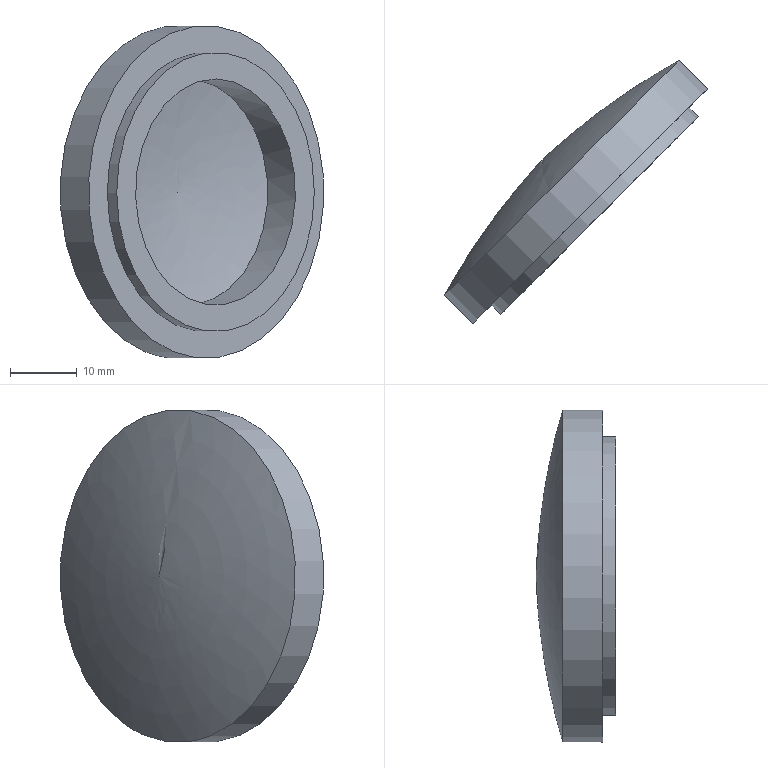Component | NX | END_CAP | 1 solid | 7 faces | box 39.6 x 39.6 x 50 mm | volume 12004 mm3 | cylinder 3 | plane 2 | spline 2 | commonest cylinder face diameters 42 x1 50 x1 34 x1
STEP:
#1=CARTESIAN_POINT('',(0.,0.,0.));
#2=DIRECTION('',(0.,0.,1.));
#3=DIRECTION('',(1.,0.,0.));
#4=AXIS2_PLACEMENT_3D('',#1,#2,#3);
#5=CARTESIAN_POINT('',(-1056.592,1684.37,243.101));
#6=VERTEX_POINT('',#5);
#7=CARTESIAN_POINT('',(-1057.899,1683.063,260.));
#8=DIRECTION('',(-0.7071,0.7071,0.));
#9=DIRECTION('',(0.07689,0.07689,-0.9941));
#10=AXIS2_PLACEMENT_3D('',#7,#8,#9);
#11=CIRCLE('',#10,17.);
#12=CARTESIAN_POINT('',(-1072.66,1668.302,257.716));
#13=DIRECTION('',(0.7071,-0.7071,0.));
#14=DIRECTION('',(0.07689,0.07689,-0.9941));
#15=AXIS2_PLACEMENT_3D('',#12,#13,#14);
#16=PLANE('',#15);
#17=CARTESIAN_POINT('',(17.,21.));
#18=CARTESIAN_POINT('',(17.,-8.445));
#19=CARTESIAN_POINT('',(-8.5,6.278));
#20=CARTESIAN_POINT('',(-34.,21.));
#21=CARTESIAN_POINT('',(-8.5,35.722));
#22=CARTESIAN_POINT('',(17.,50.445));
#23=CARTESIAN_POINT('',(17.,21.));
#24=(BOUNDED_CURVE()B_SPLINE_CURVE(2,(#17,#18,#19,#20,#21,#22,#23),.UNSPECIFIED.,.T.,.F.)B_SPLINE_CURVE_WITH_KNOTS((1,2,2,2,2,1),(-2.094,0.,2.094,4.189,6.283,8.378),.UNSPECIFIED.)CURVE()GEOMETRIC_REPRESENTATION_ITEM()RATIONAL_B_SPLINE_CURVE((1.,0.5,1.,0.5,1.,0.5,1.))REPRESENTATION_ITEM(''));
#25=(GEOMETRIC_REPRESENTATION_CONTEXT(2)PARAMETRIC_REPRESENTATION_CONTEXT()REPRESENTATION_CONTEXT('',''));
#26=DEFINITIONAL_REPRESENTATION('',(#24),#25);
#27=PCURVE('',#16,#26);
#28=CARTESIAN_POINT('',(-1057.899,1683.063,260.));
#29=DIRECTION('',(-0.7071,0.7071,0.));
#30=DIRECTION('',(-0.07689,-0.07689,0.9941));
#31=AXIS2_PLACEMENT_3D('',#28,#29,#30);
#32=CYLINDRICAL_SURFACE('',#31,17.);
#33=CARTESIAN_POINT('',(3.142,-0.));
#34=DIRECTION('',(1.,0.));
#35=VECTOR('',#34,1.);
#36=LINE('',#33,#35);
#37=(GEOMETRIC_REPRESENTATION_CONTEXT(2)PARAMETRIC_REPRESENTATION_CONTEXT()REPRESENTATION_CONTEXT('',''));
#38=DEFINITIONAL_REPRESENTATION('',(#36),#37);
#39=PCURVE('',#32,#38);
#40=SURFACE_CURVE('',#11,(#27,#39),.PCURVE_S1.);
#41=EDGE_CURVE('',#6,#6,#40,.T.);
#42=ORIENTED_EDGE('',*,*,#41,.T.);
#43=EDGE_LOOP('',(#42));
#44=FACE_BOUND('',#43,.T.);
#45=CARTESIAN_POINT('',(-1059.514,1681.448,280.875));
#46=VERTEX_POINT('',#45);
#47=CARTESIAN_POINT('',(-1057.899,1683.063,260.));
#48=DIRECTION('',(-0.7071,0.7071,0.));
#49=DIRECTION('',(-0.07689,-0.07689,0.9941));
#50=AXIS2_PLACEMENT_3D('',#47,#48,#49);
#51=CIRCLE('',#50,21.);
#52=CARTESIAN_POINT('',(-21.,21.));
#53=CARTESIAN_POINT('',(-21.,57.373));
#54=CARTESIAN_POINT('',(10.5,39.187));
#55=CARTESIAN_POINT('',(42.,21.));
#56=CARTESIAN_POINT('',(10.5,2.813));
#57=CARTESIAN_POINT('',(-21.,-15.373));
#58=CARTESIAN_POINT('',(-21.,21.));
#59=(BOUNDED_CURVE()B_SPLINE_CURVE(2,(#52,#53,#54,#55,#56,#57,#58),.UNSPECIFIED.,.T.,.F.)B_SPLINE_CURVE_WITH_KNOTS((1,2,2,2,2,1),(-2.094,0.,2.094,4.189,6.283,8.378),.UNSPECIFIED.)CURVE()GEOMETRIC_REPRESENTATION_ITEM()RATIONAL_B_SPLINE_CURVE((1.,0.5,1.,0.5,1.,0.5,1.))REPRESENTATION_ITEM(''));
#60=(GEOMETRIC_REPRESENTATION_CONTEXT(2)PARAMETRIC_REPRESENTATION_CONTEXT()REPRESENTATION_CONTEXT('',''));
#61=DEFINITIONAL_REPRESENTATION('',(#59),#60);
#62=PCURVE('',#16,#61);
#63=CARTESIAN_POINT('',(-1057.899,1683.063,260.));
#64=DIRECTION('',(-0.7071,0.7071,0.));
#65=DIRECTION('',(-0.07689,-0.07689,0.9941));
#66=AXIS2_PLACEMENT_3D('',#63,#64,#65);
#67=CYLINDRICAL_SURFACE('',#66,21.);
#68=CARTESIAN_POINT('',(0.,0.));
#69=DIRECTION('',(1.,0.));
#70=VECTOR('',#69,1.);
#71=LINE('',#68,#70);
#72=(GEOMETRIC_REPRESENTATION_CONTEXT(2)PARAMETRIC_REPRESENTATION_CONTEXT()REPRESENTATION_CONTEXT('',''));
#73=DEFINITIONAL_REPRESENTATION('',(#71),#72);
#74=PCURVE('',#67,#73);
#75=SURFACE_CURVE('',#51,(#62,#74),.PCURVE_S1.);
#76=EDGE_CURVE('',#46,#46,#75,.T.);
#77=ORIENTED_EDGE('',*,*,#76,.F.);
#78=EDGE_LOOP('',(#77));
#79=FACE_BOUND('',#78,.T.);
#80=ADVANCED_FACE('',(#44,#79),#16,.T.);
#81=ORIENTED_EDGE('',*,*,#76,.T.);
#82=CARTESIAN_POINT('',(-1060.928,1682.863,280.875));
#83=VERTEX_POINT('',#82);
#84=CARTESIAN_POINT('',(-1059.514,1681.448,280.875));
#85=CARTESIAN_POINT('',(-1060.928,1682.863,280.875));
#86=B_SPLINE_CURVE_WITH_KNOTS('',1,(#84,#85),.UNSPECIFIED.,.F.,.F.,(2,2),(0.,2.),.PIECEWISE_BEZIER_KNOTS.);
#87=CARTESIAN_POINT('',(6.283,0.));
#88=DIRECTION('',(0.,1.));
#89=VECTOR('',#88,1.);
#90=LINE('',#87,#89);
#91=(GEOMETRIC_REPRESENTATION_CONTEXT(2)PARAMETRIC_REPRESENTATION_CONTEXT()REPRESENTATION_CONTEXT('',''));
#92=DEFINITIONAL_REPRESENTATION('',(#90),#91);
#93=PCURVE('',#67,#92);
#94=CARTESIAN_POINT('',(0.,0.));
#95=DIRECTION('',(0.,1.));
#96=VECTOR('',#95,1.);
#97=LINE('',#94,#96);
#98=(GEOMETRIC_REPRESENTATION_CONTEXT(2)PARAMETRIC_REPRESENTATION_CONTEXT()REPRESENTATION_CONTEXT('',''));
#99=DEFINITIONAL_REPRESENTATION('',(#97),#98);
#100=PCURVE('',#67,#99);
#101=SEAM_CURVE('',#86,(#93,#100),.PCURVE_S1.);
#102=EDGE_CURVE('',#46,#83,#101,.T.);
#103=ORIENTED_EDGE('',*,*,#102,.T.);
#104=CARTESIAN_POINT('',(-1059.313,1684.477,260.));
#105=DIRECTION('',(-0.7071,0.7071,0.));
#106=DIRECTION('',(-0.07689,-0.07689,0.9941));
#107=AXIS2_PLACEMENT_3D('',#104,#105,#106);
#108=CIRCLE('',#107,21.);
#109=CARTESIAN_POINT('',(0.,2.));
#110=DIRECTION('',(1.,0.));
#111=VECTOR('',#110,1.);
#112=LINE('',#109,#111);
#113=(GEOMETRIC_REPRESENTATION_CONTEXT(2)PARAMETRIC_REPRESENTATION_CONTEXT()REPRESENTATION_CONTEXT('',''));
#114=DEFINITIONAL_REPRESENTATION('',(#112),#113);
#115=PCURVE('',#67,#114);
#116=CARTESIAN_POINT('',(-1076.886,1666.904,257.281));
#117=DIRECTION('',(0.7071,-0.7071,0.));
#118=DIRECTION('',(0.07689,0.07689,-0.9941));
#119=AXIS2_PLACEMENT_3D('',#116,#117,#118);
#120=PLANE('',#119);
#121=CARTESIAN_POINT('',(-21.,25.));
#122=CARTESIAN_POINT('',(-21.,61.373));
#123=CARTESIAN_POINT('',(10.5,43.187));
#124=CARTESIAN_POINT('',(42.,25.));
#125=CARTESIAN_POINT('',(10.5,6.813));
#126=CARTESIAN_POINT('',(-21.,-11.373));
#127=CARTESIAN_POINT('',(-21.,25.));
#128=(BOUNDED_CURVE()B_SPLINE_CURVE(2,(#121,#122,#123,#124,#125,#126,#127),.UNSPECIFIED.,.T.,.F.)B_SPLINE_CURVE_WITH_KNOTS((1,2,2,2,2,1),(-2.094,0.,2.094,4.189,6.283,8.378),.UNSPECIFIED.)CURVE()GEOMETRIC_REPRESENTATION_ITEM()RATIONAL_B_SPLINE_CURVE((1.,0.5,1.,0.5,1.,0.5,1.))REPRESENTATION_ITEM(''));
#129=(GEOMETRIC_REPRESENTATION_CONTEXT(2)PARAMETRIC_REPRESENTATION_CONTEXT()REPRESENTATION_CONTEXT('',''));
#130=DEFINITIONAL_REPRESENTATION('',(#128),#129);
#131=PCURVE('',#120,#130);
#132=SURFACE_CURVE('',#108,(#115,#131),.PCURVE_S1.);
#133=EDGE_CURVE('',#83,#83,#132,.T.);
#134=ORIENTED_EDGE('',*,*,#133,.F.);
#135=ORIENTED_EDGE('',*,*,#102,.F.);
#136=EDGE_LOOP('',(#81,#103,#134,#135));
#137=FACE_BOUND('',#136,.T.);
#138=ADVANCED_FACE('',(#137),#67,.T.);
#139=ORIENTED_EDGE('',*,*,#133,.T.);
#140=EDGE_LOOP('',(#139));
#141=FACE_BOUND('',#140,.T.);
#142=CARTESIAN_POINT('',(-1061.235,1682.555,284.852));
#143=VERTEX_POINT('',#142);
#144=CARTESIAN_POINT('',(-1059.313,1684.477,260.));
#145=DIRECTION('',(-0.7071,0.7071,0.));
#146=DIRECTION('',(-0.07689,-0.07689,0.9941));
#147=AXIS2_PLACEMENT_3D('',#144,#145,#146);
#148=CIRCLE('',#147,25.);
#149=CARTESIAN_POINT('',(-25.,25.));
#150=CARTESIAN_POINT('',(-25.,68.301));
#151=CARTESIAN_POINT('',(12.5,46.651));
#152=CARTESIAN_POINT('',(50.,25.));
#153=CARTESIAN_POINT('',(12.5,3.349));
#154=CARTESIAN_POINT('',(-25.,-18.301));
#155=CARTESIAN_POINT('',(-25.,25.));
#156=(BOUNDED_CURVE()B_SPLINE_CURVE(2,(#149,#150,#151,#152,#153,#154,#155),.UNSPECIFIED.,.T.,.F.)B_SPLINE_CURVE_WITH_KNOTS((1,2,2,2,2,1),(-2.094,0.,2.094,4.189,6.283,8.378),.UNSPECIFIED.)CURVE()GEOMETRIC_REPRESENTATION_ITEM()RATIONAL_B_SPLINE_CURVE((1.,0.5,1.,0.5,1.,0.5,1.))REPRESENTATION_ITEM(''));
#157=(GEOMETRIC_REPRESENTATION_CONTEXT(2)PARAMETRIC_REPRESENTATION_CONTEXT()REPRESENTATION_CONTEXT('',''));
#158=DEFINITIONAL_REPRESENTATION('',(#156),#157);
#159=PCURVE('',#120,#158);
#160=CARTESIAN_POINT('',(-1057.899,1683.063,260.));
#161=DIRECTION('',(-0.7071,0.7071,0.));
#162=DIRECTION('',(-0.07689,-0.07689,0.9941));
#163=AXIS2_PLACEMENT_3D('',#160,#161,#162);
#164=CYLINDRICAL_SURFACE('',#163,25.);
#165=CARTESIAN_POINT('',(0.,2.));
#166=DIRECTION('',(1.,0.));
#167=VECTOR('',#166,1.);
#168=LINE('',#165,#167);
#169=(GEOMETRIC_REPRESENTATION_CONTEXT(2)PARAMETRIC_REPRESENTATION_CONTEXT()REPRESENTATION_CONTEXT('',''));
#170=DEFINITIONAL_REPRESENTATION('',(#168),#169);
#171=PCURVE('',#164,#170);
#172=SURFACE_CURVE('',#148,(#159,#171),.PCURVE_S1.);
#173=EDGE_CURVE('',#143,#143,#172,.T.);
#174=ORIENTED_EDGE('',*,*,#173,.F.);
#175=EDGE_LOOP('',(#174));
#176=FACE_BOUND('',#175,.T.);
#177=ADVANCED_FACE('',(#141,#176),#120,.T.);
#178=ORIENTED_EDGE('',*,*,#173,.T.);
#179=CARTESIAN_POINT('',(-1065.478,1686.798,284.852));
#180=VERTEX_POINT('',#179);
#181=CARTESIAN_POINT('',(-1061.235,1682.555,284.852));
#182=CARTESIAN_POINT('',(-1065.478,1686.798,284.852));
#183=B_SPLINE_CURVE_WITH_KNOTS('',1,(#181,#182),.UNSPECIFIED.,.F.,.F.,(2,2),(2.,8.),.PIECEWISE_BEZIER_KNOTS.);
#184=CARTESIAN_POINT('',(6.283,0.));
#185=DIRECTION('',(0.,1.));
#186=VECTOR('',#185,1.);
#187=LINE('',#184,#186);
#188=(GEOMETRIC_REPRESENTATION_CONTEXT(2)PARAMETRIC_REPRESENTATION_CONTEXT()REPRESENTATION_CONTEXT('',''));
#189=DEFINITIONAL_REPRESENTATION('',(#187),#188);
#190=PCURVE('',#164,#189);
#191=CARTESIAN_POINT('',(0.,0.));
#192=DIRECTION('',(0.,1.));
#193=VECTOR('',#192,1.);
#194=LINE('',#191,#193);
#195=(GEOMETRIC_REPRESENTATION_CONTEXT(2)PARAMETRIC_REPRESENTATION_CONTEXT()REPRESENTATION_CONTEXT('',''));
#196=DEFINITIONAL_REPRESENTATION('',(#194),#195);
#197=PCURVE('',#164,#196);
#198=SEAM_CURVE('',#183,(#190,#197),.PCURVE_S1.);
#199=EDGE_CURVE('',#143,#180,#198,.T.);
#200=ORIENTED_EDGE('',*,*,#199,.T.);
#201=CARTESIAN_POINT('',(-1063.556,1688.72,260.));
#202=DIRECTION('',(-0.7071,0.7071,0.));
#203=DIRECTION('',(-0.07689,-0.07689,0.9941));
#204=AXIS2_PLACEMENT_3D('',#201,#202,#203);
#205=CIRCLE('',#204,25.);
#206=CARTESIAN_POINT('',(0.,8.));
#207=DIRECTION('',(1.,0.));
#208=VECTOR('',#207,1.);
#209=LINE('',#206,#208);
#210=(GEOMETRIC_REPRESENTATION_CONTEXT(2)PARAMETRIC_REPRESENTATION_CONTEXT()REPRESENTATION_CONTEXT('',''));
#211=DEFINITIONAL_REPRESENTATION('',(#209),#210);
#212=PCURVE('',#164,#211);
#213=CARTESIAN_POINT('',(-1066.384,1691.548,260.));
#214=CARTESIAN_POINT('',(-1066.384,1691.548,260.));
#215=CARTESIAN_POINT('',(-1066.384,1691.548,260.));
#216=CARTESIAN_POINT('',(-1066.384,1691.548,260.));
#217=CARTESIAN_POINT('',(-1066.384,1691.548,260.));
#218=CARTESIAN_POINT('',(-1066.384,1691.548,260.));
#219=CARTESIAN_POINT('',(-1066.384,1691.548,260.));
#220=CARTESIAN_POINT('',(-1066.846,1690.706,268.43));
#221=CARTESIAN_POINT('',(-1054.924,1702.628,270.275));
#222=CARTESIAN_POINT('',(-1053.62,1703.932,253.414));
#223=CARTESIAN_POINT('',(-1065.542,1692.01,251.57));
#224=CARTESIAN_POINT('',(-1077.464,1680.088,249.725));
#225=CARTESIAN_POINT('',(-1078.768,1678.784,266.586));
#226=CARTESIAN_POINT('',(-1066.846,1690.706,268.43));
#227=CARTESIAN_POINT('',(-1066.542,1689.114,276.759));
#228=CARTESIAN_POINT('',(-1042.842,1712.814,280.425));
#229=CARTESIAN_POINT('',(-1040.249,1715.407,246.908));
#230=CARTESIAN_POINT('',(-1063.95,1691.706,243.241));
#231=CARTESIAN_POINT('',(-1087.65,1668.006,239.575));
#232=CARTESIAN_POINT('',(-1090.243,1665.413,273.092));
#233=CARTESIAN_POINT('',(-1066.542,1689.114,276.759));
#234=CARTESIAN_POINT('',(-1065.478,1686.798,284.852));
#235=CARTESIAN_POINT('',(-1030.332,1721.943,290.289));
#236=CARTESIAN_POINT('',(-1026.488,1725.788,240.585));
#237=CARTESIAN_POINT('',(-1061.634,1690.642,235.148));
#238=CARTESIAN_POINT('',(-1096.779,1655.497,229.711));
#239=CARTESIAN_POINT('',(-1100.624,1651.652,279.415));
#240=CARTESIAN_POINT('',(-1065.478,1686.798,284.852));
#241=(BOUNDED_SURFACE()B_SPLINE_SURFACE(3,3,((#213,#214,#215,#216,#217,#218,#219),(#220,#221,#222,#223,#224,#225,#226),(#227,#228,#229,#230,#231,#232,#233),(#234,#235,#236,#237,#238,#239,#240)),.UNSPECIFIED.,.F.,.T.,.F.)B_SPLINE_SURFACE_WITH_KNOTS((4,4),(1,3,3,3,1),(0.,1.),(-0.5,0.,0.5,1.,1.5),.UNSPECIFIED.)GEOMETRIC_REPRESENTATION_ITEM()RATIONAL_B_SPLINE_SURFACE(((1.,0.3333,0.3333,1.,0.3333,0.3333,1.),(0.9946,0.3315,0.3315,0.9946,0.3315,0.3315,0.9946),(0.9946,0.3315,0.3315,0.9946,0.3315,0.3315,0.9946),(1.,0.3333,0.3333,1.,0.3333,0.3333,1.)))REPRESENTATION_ITEM('')SURFACE());
#242=CARTESIAN_POINT('',(1.,0.));
#243=CARTESIAN_POINT('',(1.,0.02352));
#244=CARTESIAN_POINT('',(1.,0.06491));
#245=CARTESIAN_POINT('',(1.,0.1146));
#246=CARTESIAN_POINT('',(1.,0.1575));
#247=CARTESIAN_POINT('',(1.,0.196));
#248=CARTESIAN_POINT('',(1.,0.2322));
#249=CARTESIAN_POINT('',(1.,0.2678));
#250=CARTESIAN_POINT('',(1.,0.304));
#251=CARTESIAN_POINT('',(1.,0.3425));
#252=CARTESIAN_POINT('',(1.,0.3856));
#253=CARTESIAN_POINT('',(1.,0.4343));
#254=CARTESIAN_POINT('',(1.,0.5));
#255=CARTESIAN_POINT('',(1.,0.5657));
#256=CARTESIAN_POINT('',(1.,0.6144));
#257=CARTESIAN_POINT('',(1.,0.6575));
#258=CARTESIAN_POINT('',(1.,0.696));
#259=CARTESIAN_POINT('',(1.,0.7322));
#260=CARTESIAN_POINT('',(1.,0.7678));
#261=CARTESIAN_POINT('',(1.,0.804));
#262=CARTESIAN_POINT('',(1.,0.8425));
#263=CARTESIAN_POINT('',(1.,0.8854));
#264=CARTESIAN_POINT('',(1.,0.9351));
#265=CARTESIAN_POINT('',(1.,0.9765));
#266=CARTESIAN_POINT('',(1.,1.));
#267=B_SPLINE_CURVE_WITH_KNOTS('',3,(#242,#243,#244,#245,#246,#247,#248,#249,#250,#251,#252,#253,#254,#255,#256,#257,#258,#259,#260,#261,#262,#263,#264,#265,#266),.UNSPECIFIED.,.F.,.F.,(4,1,1,1,1,1,1,1,1,1,1,1,1,1,1,1,1,1,1,1,1,1,4),(0.,0.2856,0.5712,0.8568,1.142,1.428,1.714,1.999,2.285,2.57,2.856,3.142,3.427,3.713,3.998,4.284,4.57,4.855,5.141,5.426,5.712,5.998,6.283),.QUASI_UNIFORM_KNOTS.);
#268=(GEOMETRIC_REPRESENTATION_CONTEXT(2)PARAMETRIC_REPRESENTATION_CONTEXT()REPRESENTATION_CONTEXT('',''));
#269=DEFINITIONAL_REPRESENTATION('',(#267),#268);
#270=PCURVE('',#241,#269);
#271=SURFACE_CURVE('',#205,(#212,#270),.PCURVE_S1.);
#272=EDGE_CURVE('',#180,#180,#271,.T.);
#273=ORIENTED_EDGE('',*,*,#272,.F.);
#274=ORIENTED_EDGE('',*,*,#199,.F.);
#275=EDGE_LOOP('',(#178,#200,#273,#274));
#276=FACE_BOUND('',#275,.T.);
#277=ADVANCED_FACE('',(#276),#164,.T.);
#278=ORIENTED_EDGE('',*,*,#272,.T.);
#279=CARTESIAN_POINT('',(-1066.384,1691.548,260.));
#280=VERTEX_POINT('',#279);
#281=CARTESIAN_POINT('',(-1066.384,1691.548,260.));
#282=CARTESIAN_POINT('',(-1066.846,1690.706,268.43));
#283=CARTESIAN_POINT('',(-1066.542,1689.114,276.759));
#284=CARTESIAN_POINT('',(-1065.478,1686.798,284.852));
#285=(BOUNDED_CURVE()B_SPLINE_CURVE(3,(#281,#282,#283,#284),.UNSPECIFIED.,.F.,.F.)B_SPLINE_CURVE_WITH_KNOTS((4,4),(0.,1.),.PIECEWISE_BEZIER_KNOTS.)CURVE()GEOMETRIC_REPRESENTATION_ITEM()RATIONAL_B_SPLINE_CURVE((1.,0.9946,0.9946,1.))REPRESENTATION_ITEM(''));
#286=CARTESIAN_POINT('',(0.,1.));
#287=DIRECTION('',(1.,0.));
#288=VECTOR('',#287,1.);
#289=LINE('',#286,#288);
#290=(GEOMETRIC_REPRESENTATION_CONTEXT(2)PARAMETRIC_REPRESENTATION_CONTEXT()REPRESENTATION_CONTEXT('',''));
#291=DEFINITIONAL_REPRESENTATION('',(#289),#290);
#292=PCURVE('',#241,#291);
#293=CARTESIAN_POINT('',(0.,0.));
#294=DIRECTION('',(1.,0.));
#295=VECTOR('',#294,1.);
#296=LINE('',#293,#295);
#297=(GEOMETRIC_REPRESENTATION_CONTEXT(2)PARAMETRIC_REPRESENTATION_CONTEXT()REPRESENTATION_CONTEXT('',''));
#298=DEFINITIONAL_REPRESENTATION('',(#296),#297);
#299=PCURVE('',#241,#298);
#300=SEAM_CURVE('',#285,(#292,#299),.PCURVE_S1.);
#301=EDGE_CURVE('',#280,#180,#300,.T.);
#302=ORIENTED_EDGE('',*,*,#301,.F.);
#303=ORIENTED_EDGE('',*,*,#301,.T.);
#304=EDGE_LOOP('',(#278,#302,#303));
#305=FACE_BOUND('',#304,.T.);
#306=ADVANCED_FACE('',(#305),#241,.T.);
#307=ORIENTED_EDGE('',*,*,#41,.T.);
#308=CARTESIAN_POINT('',(-1060.769,1688.547,243.101));
#309=VERTEX_POINT('',#308);
#310=CARTESIAN_POINT('',(-1056.592,1684.37,243.101));
#311=CARTESIAN_POINT('',(-1060.769,1688.547,243.101));
#312=B_SPLINE_CURVE_WITH_KNOTS('',1,(#310,#311),.UNSPECIFIED.,.F.,.F.,(2,2),(-0.,5.907),.PIECEWISE_BEZIER_KNOTS.);
#313=CARTESIAN_POINT('',(9.425,0.));
#314=DIRECTION('',(0.,1.));
#315=VECTOR('',#314,1.);
#316=LINE('',#313,#315);
#317=(GEOMETRIC_REPRESENTATION_CONTEXT(2)PARAMETRIC_REPRESENTATION_CONTEXT()REPRESENTATION_CONTEXT('',''));
#318=DEFINITIONAL_REPRESENTATION('',(#316),#317);
#319=PCURVE('',#32,#318);
#320=CARTESIAN_POINT('',(3.142,0.));
#321=DIRECTION('',(0.,1.));
#322=VECTOR('',#321,1.);
#323=LINE('',#320,#322);
#324=(GEOMETRIC_REPRESENTATION_CONTEXT(2)PARAMETRIC_REPRESENTATION_CONTEXT()REPRESENTATION_CONTEXT('',''));
#325=DEFINITIONAL_REPRESENTATION('',(#323),#324);
#326=PCURVE('',#32,#325);
#327=SEAM_CURVE('',#312,(#319,#326),.PCURVE_S1.);
#328=EDGE_CURVE('',#6,#309,#327,.T.);
#329=ORIENTED_EDGE('',*,*,#328,.T.);
#330=CARTESIAN_POINT('',(-1063.383,1685.933,276.899));
#331=VERTEX_POINT('',#330);
#332=CARTESIAN_POINT('',(-1062.076,1687.24,260.));
#333=DIRECTION('',(0.7071,-0.7071,0.));
#334=DIRECTION('',(0.07689,0.07689,-0.9941));
#335=AXIS2_PLACEMENT_3D('',#332,#333,#334);
#336=CIRCLE('',#335,17.);
#337=CARTESIAN_POINT('',(9.425,5.907));
#338=DIRECTION('',(-1.,0.));
#339=VECTOR('',#338,1.);
#340=LINE('',#337,#339);
#341=(GEOMETRIC_REPRESENTATION_CONTEXT(2)PARAMETRIC_REPRESENTATION_CONTEXT()REPRESENTATION_CONTEXT('',''));
#342=DEFINITIONAL_REPRESENTATION('',(#340),#341);
#343=PCURVE('',#32,#342);
#344=CARTESIAN_POINT('',(-1063.383,1685.933,276.899));
#345=CARTESIAN_POINT('',(-1039.484,1709.832,280.596));
#346=CARTESIAN_POINT('',(-1036.87,1712.446,246.798));
#347=CARTESIAN_POINT('',(-1060.769,1688.547,243.101));
#348=CARTESIAN_POINT('',(-1084.668,1664.648,239.404));
#349=CARTESIAN_POINT('',(-1087.282,1662.034,273.202));
#350=CARTESIAN_POINT('',(-1063.383,1685.933,276.899));
#351=CARTESIAN_POINT('',(-1063.803,1687.214,271.336));
#352=CARTESIAN_POINT('',(-1047.772,1703.245,273.816));
#353=CARTESIAN_POINT('',(-1046.019,1704.998,251.144));
#354=CARTESIAN_POINT('',(-1062.05,1688.967,248.664));
#355=CARTESIAN_POINT('',(-1078.081,1672.936,246.184));
#356=CARTESIAN_POINT('',(-1079.834,1671.183,268.856));
#357=CARTESIAN_POINT('',(-1063.803,1687.214,271.336));
#358=CARTESIAN_POINT('',(-1063.861,1688.145,265.688));
#359=CARTESIAN_POINT('',(-1055.817,1696.188,266.932));
#360=CARTESIAN_POINT('',(-1054.937,1697.068,255.557));
#361=CARTESIAN_POINT('',(-1062.981,1689.025,254.312));
#362=CARTESIAN_POINT('',(-1071.024,1680.981,253.068));
#363=CARTESIAN_POINT('',(-1071.904,1680.101,264.443));
#364=CARTESIAN_POINT('',(-1063.861,1688.145,265.688));
#365=CARTESIAN_POINT('',(-1063.554,1688.718,260.));
#366=CARTESIAN_POINT('',(-1063.554,1688.718,260.));
#367=CARTESIAN_POINT('',(-1063.554,1688.718,260.));
#368=CARTESIAN_POINT('',(-1063.554,1688.718,260.));
#369=CARTESIAN_POINT('',(-1063.554,1688.718,260.));
#370=CARTESIAN_POINT('',(-1063.554,1688.718,260.));
#371=CARTESIAN_POINT('',(-1063.554,1688.718,260.));
#372=(BOUNDED_SURFACE()B_SPLINE_SURFACE(3,3,((#344,#345,#346,#347,#348,#349,#350),(#351,#352,#353,#354,#355,#356,#357),(#358,#359,#360,#361,#362,#363,#364),(#365,#366,#367,#368,#369,#370,#371)),.UNSPECIFIED.,.F.,.T.,.F.)B_SPLINE_SURFACE_WITH_KNOTS((4,4),(1,3,3,3,1),(0.,1.),(-0.5,0.,0.5,1.,1.5),.UNSPECIFIED.)GEOMETRIC_REPRESENTATION_ITEM()RATIONAL_B_SPLINE_SURFACE(((1.,0.3333,0.3333,1.,0.3333,0.3333,1.),(0.9973,0.3324,0.3324,0.9973,0.3324,0.3324,0.9973),(0.9973,0.3324,0.3324,0.9973,0.3324,0.3324,0.9973),(1.,0.3333,0.3333,1.,0.3333,0.3333,1.)))REPRESENTATION_ITEM('')SURFACE());
#373=CARTESIAN_POINT('',(0.,0.5));
#374=CARTESIAN_POINT('',(0.,0.4765));
#375=CARTESIAN_POINT('',(0.,0.4351));
#376=CARTESIAN_POINT('',(0.,0.3854));
#377=CARTESIAN_POINT('',(0.,0.3425));
#378=CARTESIAN_POINT('',(0.,0.304));
#379=CARTESIAN_POINT('',(0.,0.2678));
#380=CARTESIAN_POINT('',(0.,0.2322));
#381=CARTESIAN_POINT('',(0.,0.196));
#382=CARTESIAN_POINT('',(0.,0.1575));
#383=CARTESIAN_POINT('',(0.,0.1144));
#384=CARTESIAN_POINT('',(0.,0.06567));
#385=CARTESIAN_POINT('',(0.,-0.));
#386=CARTESIAN_POINT('',(0.,-0.06567));
#387=CARTESIAN_POINT('',(-0.,-0.1144));
#388=CARTESIAN_POINT('',(-0.,-0.1575));
#389=CARTESIAN_POINT('',(-0.,-0.196));
#390=CARTESIAN_POINT('',(-0.,-0.2322));
#391=CARTESIAN_POINT('',(-0.,-0.2678));
#392=CARTESIAN_POINT('',(-0.,-0.304));
#393=CARTESIAN_POINT('',(-0.,-0.3425));
#394=CARTESIAN_POINT('',(-0.,-0.3854));
#395=CARTESIAN_POINT('',(-0.,-0.4351));
#396=CARTESIAN_POINT('',(-0.,-0.4765));
#397=CARTESIAN_POINT('',(0.,-0.5));
#398=B_SPLINE_CURVE_WITH_KNOTS('',3,(#373,#374,#375,#376,#377,#378,#379,#380,#381,#382,#383,#384,#385,#386,#387,#388,#389,#390,#391,#392,#393,#394,#395,#396,#397),.UNSPECIFIED.,.F.,.F.,(4,1,1,1,1,1,1,1,1,1,1,1,1,1,1,1,1,1,1,1,1,1,4),(0.,0.2856,0.5712,0.8568,1.142,1.428,1.714,1.999,2.285,2.57,2.856,3.142,3.427,3.713,3.998,4.284,4.57,4.855,5.141,5.426,5.712,5.998,6.283),.QUASI_UNIFORM_KNOTS.);
#399=(GEOMETRIC_REPRESENTATION_CONTEXT(2)PARAMETRIC_REPRESENTATION_CONTEXT()REPRESENTATION_CONTEXT('',''));
#400=DEFINITIONAL_REPRESENTATION('',(#398),#399);
#401=PCURVE('',#372,#400);
#402=SURFACE_CURVE('',#336,(#343,#401),.PCURVE_S1.);
#403=EDGE_CURVE('',#309,#331,#402,.T.);
#404=ORIENTED_EDGE('',*,*,#403,.T.);
#405=CARTESIAN_POINT('',(-1062.076,1687.24,260.));
#406=DIRECTION('',(0.7071,-0.7071,0.));
#407=DIRECTION('',(0.07689,0.07689,-0.9941));
#408=AXIS2_PLACEMENT_3D('',#405,#406,#407);
#409=CIRCLE('',#408,17.);
#410=CARTESIAN_POINT('',(9.425,5.907));
#411=DIRECTION('',(-1.,0.));
#412=VECTOR('',#411,1.);
#413=LINE('',#410,#412);
#414=(GEOMETRIC_REPRESENTATION_CONTEXT(2)PARAMETRIC_REPRESENTATION_CONTEXT()REPRESENTATION_CONTEXT('',''));
#415=DEFINITIONAL_REPRESENTATION('',(#413),#414);
#416=PCURVE('',#32,#415);
#417=CARTESIAN_POINT('',(0.,1.5));
#418=CARTESIAN_POINT('',(0.,1.476));
#419=CARTESIAN_POINT('',(0.,1.435));
#420=CARTESIAN_POINT('',(0.,1.385));
#421=CARTESIAN_POINT('',(0.,1.343));
#422=CARTESIAN_POINT('',(0.,1.304));
#423=CARTESIAN_POINT('',(0.,1.268));
#424=CARTESIAN_POINT('',(0.,1.232));
#425=CARTESIAN_POINT('',(0.,1.196));
#426=CARTESIAN_POINT('',(0.,1.158));
#427=CARTESIAN_POINT('',(0.,1.114));
#428=CARTESIAN_POINT('',(0.,1.066));
#429=CARTESIAN_POINT('',(0.,1.));
#430=CARTESIAN_POINT('',(0.,0.9343));
#431=CARTESIAN_POINT('',(-0.,0.8856));
#432=CARTESIAN_POINT('',(-0.,0.8425));
#433=CARTESIAN_POINT('',(-0.,0.804));
#434=CARTESIAN_POINT('',(-0.,0.7678));
#435=CARTESIAN_POINT('',(-0.,0.7322));
#436=CARTESIAN_POINT('',(-0.,0.696));
#437=CARTESIAN_POINT('',(-0.,0.6575));
#438=CARTESIAN_POINT('',(-0.,0.6146));
#439=CARTESIAN_POINT('',(-0.,0.5649));
#440=CARTESIAN_POINT('',(-0.,0.5235));
#441=CARTESIAN_POINT('',(0.,0.5));
#442=B_SPLINE_CURVE_WITH_KNOTS('',3,(#417,#418,#419,#420,#421,#422,#423,#424,#425,#426,#427,#428,#429,#430,#431,#432,#433,#434,#435,#436,#437,#438,#439,#440,#441),.UNSPECIFIED.,.F.,.F.,(4,1,1,1,1,1,1,1,1,1,1,1,1,1,1,1,1,1,1,1,1,1,4),(0.,0.2856,0.5712,0.8568,1.142,1.428,1.714,1.999,2.285,2.57,2.856,3.142,3.427,3.713,3.998,4.284,4.57,4.855,5.141,5.426,5.712,5.998,6.283),.QUASI_UNIFORM_KNOTS.);
#443=(GEOMETRIC_REPRESENTATION_CONTEXT(2)PARAMETRIC_REPRESENTATION_CONTEXT()REPRESENTATION_CONTEXT('',''));
#444=DEFINITIONAL_REPRESENTATION('',(#442),#443);
#445=PCURVE('',#372,#444);
#446=SURFACE_CURVE('',#409,(#416,#445),.PCURVE_S1.);
#447=EDGE_CURVE('',#331,#309,#446,.T.);
#448=ORIENTED_EDGE('',*,*,#447,.T.);
#449=ORIENTED_EDGE('',*,*,#328,.F.);
#450=EDGE_LOOP('',(#307,#329,#404,#448,#449));
#451=FACE_BOUND('',#450,.F.);
#452=ADVANCED_FACE('',(#451),#32,.F.);
#453=ORIENTED_EDGE('',*,*,#403,.T.);
#454=CARTESIAN_POINT('',(-1063.554,1688.718,260.));
#455=VERTEX_POINT('',#454);
#456=CARTESIAN_POINT('',(-1063.383,1685.933,276.899));
#457=CARTESIAN_POINT('',(-1063.803,1687.214,271.336));
#458=CARTESIAN_POINT('',(-1063.861,1688.145,265.688));
#459=CARTESIAN_POINT('',(-1063.554,1688.718,260.));
#460=(BOUNDED_CURVE()B_SPLINE_CURVE(3,(#456,#457,#458,#459),.UNSPECIFIED.,.F.,.F.)B_SPLINE_CURVE_WITH_KNOTS((4,4),(0.,1.),.PIECEWISE_BEZIER_KNOTS.)CURVE()GEOMETRIC_REPRESENTATION_ITEM()RATIONAL_B_SPLINE_CURVE((1.,0.9973,0.9973,1.))REPRESENTATION_ITEM(''));
#461=CARTESIAN_POINT('',(0.,0.));
#462=DIRECTION('',(1.,0.));
#463=VECTOR('',#462,1.);
#464=LINE('',#461,#463);
#465=(GEOMETRIC_REPRESENTATION_CONTEXT(2)PARAMETRIC_REPRESENTATION_CONTEXT()REPRESENTATION_CONTEXT('',''));
#466=DEFINITIONAL_REPRESENTATION('',(#464),#465);
#467=PCURVE('',#372,#466);
#468=CARTESIAN_POINT('',(0.,1.));
#469=DIRECTION('',(1.,0.));
#470=VECTOR('',#469,1.);
#471=LINE('',#468,#470);
#472=(GEOMETRIC_REPRESENTATION_CONTEXT(2)PARAMETRIC_REPRESENTATION_CONTEXT()REPRESENTATION_CONTEXT('',''));
#473=DEFINITIONAL_REPRESENTATION('',(#471),#472);
#474=PCURVE('',#372,#473);
#475=SEAM_CURVE('',#460,(#467,#474),.PCURVE_S1.);
#476=EDGE_CURVE('',#331,#455,#475,.T.);
#477=ORIENTED_EDGE('',*,*,#476,.T.);
#478=ORIENTED_EDGE('',*,*,#476,.F.);
#479=ORIENTED_EDGE('',*,*,#447,.T.);
#480=EDGE_LOOP('',(#453,#477,#478,#479));
#481=FACE_BOUND('',#480,.T.);
#482=ADVANCED_FACE('',(#481),#372,.T.);
#483=CLOSED_SHELL('',(#80,#138,#177,#277,#306,#452,#482));
#484=MANIFOLD_SOLID_BREP('',#483);
#485=(LENGTH_UNIT()NAMED_UNIT(*)SI_UNIT(.MILLI.,.METRE.));
#486=UNCERTAINTY_MEASURE_WITH_UNIT(LENGTH_MEASURE(0.01),#485,'','');
#487=(NAMED_UNIT(*)PLANE_ANGLE_UNIT()SI_UNIT($,.RADIAN.));
#488=(NAMED_UNIT(*)SI_UNIT($,.STERADIAN.)SOLID_ANGLE_UNIT());
#489=(GEOMETRIC_REPRESENTATION_CONTEXT(3)GLOBAL_UNCERTAINTY_ASSIGNED_CONTEXT((#486))GLOBAL_UNIT_ASSIGNED_CONTEXT((#485,#487,#488))REPRESENTATION_CONTEXT('',''));
#490=ADVANCED_BREP_SHAPE_REPRESENTATION('',(#4,#484),#489);